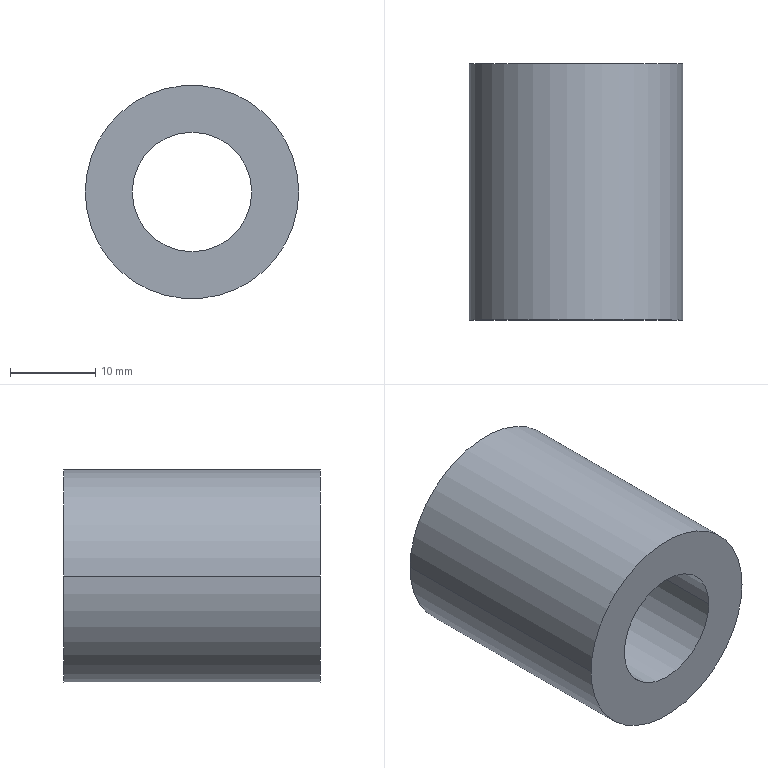Component | SolidWorks | UpperBushing-1 | 1 solid | 6 faces | box 25 x 30 x 25 mm | volume 10108 mm3 | cylinder 4 | plane 2 | commonest cylinder face diameters 14 x2 25 x2
build123d program:
from build123d import *

# Parameters (mm, degrees)
SKETCH1_R           = 12.5
SKETCH1_R_2         = 7
BOSS_EXTRUDE1_DEPTH = 30


with BuildPart() as part:
    # Sketch1 → Boss-Extrude1 (new body)
    with BuildSketch(Plane.XY):
        with Locations((-75, 62.5)):
            Circle(SKETCH1_R)
        with Locations((-75, 62.5)):
            Circle(SKETCH1_R_2, mode=Mode.SUBTRACT)
    extrude(amount=-BOSS_EXTRUDE1_DEPTH)


solid = part.part

# Placed as in the assembly
solid = solid.moved(Location((0, 170.565, -125), (90, 0, 0)))
STEP:
#1=CARTESIAN_POINT('',(-3.228,6.715,-2.461));
#2=VERTEX_POINT('',#1);
#3=CARTESIAN_POINT('',(-2.677,6.715,-2.461));
#4=VERTEX_POINT('',#3);
#5=CARTESIAN_POINT('',(-2.953,6.715,-2.461));
#6=DIRECTION('',(0.,1.,0.));
#7=DIRECTION('',(1.,0.,0.));
#8=AXIS2_PLACEMENT_3D('',#5,#6,#7);
#9=CIRCLE('',#8,0.2756);
#10=EDGE_CURVE('',#2,#4,#9,.T.);
#11=ORIENTED_EDGE('',*,*,#10,.F.);
#12=CARTESIAN_POINT('',(-3.228,7.896,-2.461));
#13=VERTEX_POINT('',#12);
#14=CARTESIAN_POINT('',(-3.228,6.715,-2.461));
#15=DIRECTION('',(0.,1.,0.));
#16=VECTOR('',#15,39.37);
#17=LINE('',#14,#16);
#18=EDGE_CURVE('',#2,#13,#17,.T.);
#19=ORIENTED_EDGE('',*,*,#18,.T.);
#20=CARTESIAN_POINT('',(-2.677,7.896,-2.461));
#21=VERTEX_POINT('',#20);
#22=CARTESIAN_POINT('',(-2.953,7.896,-2.461));
#23=DIRECTION('',(0.,1.,0.));
#24=DIRECTION('',(1.,0.,0.));
#25=AXIS2_PLACEMENT_3D('',#22,#23,#24);
#26=CIRCLE('',#25,0.2756);
#27=EDGE_CURVE('',#13,#21,#26,.T.);
#28=ORIENTED_EDGE('',*,*,#27,.T.);
#29=CARTESIAN_POINT('',(-2.677,6.715,-2.461));
#30=DIRECTION('',(0.,1.,0.));
#31=VECTOR('',#30,39.37);
#32=LINE('',#29,#31);
#33=EDGE_CURVE('',#4,#21,#32,.T.);
#34=ORIENTED_EDGE('',*,*,#33,.F.);
#35=EDGE_LOOP('',(#11,#19,#28,#34));
#36=FACE_OUTER_BOUND('',#35,.T.);
#37=CARTESIAN_POINT('',(-2.953,6.715,-2.461));
#38=DIRECTION('',(0.,1.,0.));
#39=DIRECTION('',(1.,0.,0.));
#40=AXIS2_PLACEMENT_3D('',#37,#38,#39);
#41=CYLINDRICAL_SURFACE('',#40,0.2756);
#42=ADVANCED_FACE('',(#36),#41,.F.);
#43=CARTESIAN_POINT('',(-2.461,6.715,-2.461));
#44=VERTEX_POINT('',#43);
#45=CARTESIAN_POINT('',(-3.445,6.715,-2.461));
#46=VERTEX_POINT('',#45);
#47=CARTESIAN_POINT('',(-2.953,6.715,-2.461));
#48=DIRECTION('',(0.,1.,0.));
#49=DIRECTION('',(1.,0.,0.));
#50=AXIS2_PLACEMENT_3D('',#47,#48,#49);
#51=CIRCLE('',#50,0.4921);
#52=EDGE_CURVE('',#44,#46,#51,.T.);
#53=ORIENTED_EDGE('',*,*,#52,.T.);
#54=CARTESIAN_POINT('',(-3.445,7.896,-2.461));
#55=VERTEX_POINT('',#54);
#56=CARTESIAN_POINT('',(-3.445,6.715,-2.461));
#57=DIRECTION('',(0.,1.,0.));
#58=VECTOR('',#57,39.37);
#59=LINE('',#56,#58);
#60=EDGE_CURVE('',#46,#55,#59,.T.);
#61=ORIENTED_EDGE('',*,*,#60,.T.);
#62=CARTESIAN_POINT('',(-2.461,7.896,-2.461));
#63=VERTEX_POINT('',#62);
#64=CARTESIAN_POINT('',(-2.953,7.896,-2.461));
#65=DIRECTION('',(0.,1.,0.));
#66=DIRECTION('',(1.,0.,0.));
#67=AXIS2_PLACEMENT_3D('',#64,#65,#66);
#68=CIRCLE('',#67,0.4921);
#69=EDGE_CURVE('',#63,#55,#68,.T.);
#70=ORIENTED_EDGE('',*,*,#69,.F.);
#71=CARTESIAN_POINT('',(-2.461,6.715,-2.461));
#72=DIRECTION('',(0.,1.,0.));
#73=VECTOR('',#72,39.37);
#74=LINE('',#71,#73);
#75=EDGE_CURVE('',#44,#63,#74,.T.);
#76=ORIENTED_EDGE('',*,*,#75,.F.);
#77=EDGE_LOOP('',(#53,#61,#70,#76));
#78=FACE_OUTER_BOUND('',#77,.T.);
#79=CARTESIAN_POINT('',(-2.953,6.715,-2.461));
#80=DIRECTION('',(0.,1.,0.));
#81=DIRECTION('',(1.,0.,0.));
#82=AXIS2_PLACEMENT_3D('',#79,#80,#81);
#83=CYLINDRICAL_SURFACE('',#82,0.4921);
#84=ADVANCED_FACE('',(#78),#83,.T.);
#85=ORIENTED_EDGE('',*,*,#60,.F.);
#86=CARTESIAN_POINT('',(-2.953,6.715,-2.461));
#87=DIRECTION('',(0.,1.,0.));
#88=DIRECTION('',(1.,0.,0.));
#89=AXIS2_PLACEMENT_3D('',#86,#87,#88);
#90=CIRCLE('',#89,0.4921);
#91=EDGE_CURVE('',#46,#44,#90,.T.);
#92=ORIENTED_EDGE('',*,*,#91,.T.);
#93=ORIENTED_EDGE('',*,*,#75,.T.);
#94=CARTESIAN_POINT('',(-2.953,7.896,-2.461));
#95=DIRECTION('',(0.,1.,0.));
#96=DIRECTION('',(1.,0.,0.));
#97=AXIS2_PLACEMENT_3D('',#94,#95,#96);
#98=CIRCLE('',#97,0.4921);
#99=EDGE_CURVE('',#55,#63,#98,.T.);
#100=ORIENTED_EDGE('',*,*,#99,.F.);
#101=EDGE_LOOP('',(#85,#92,#93,#100));
#102=FACE_OUTER_BOUND('',#101,.T.);
#103=CARTESIAN_POINT('',(-2.953,6.715,-2.461));
#104=DIRECTION('',(0.,1.,0.));
#105=DIRECTION('',(1.,0.,0.));
#106=AXIS2_PLACEMENT_3D('',#103,#104,#105);
#107=CYLINDRICAL_SURFACE('',#106,0.4921);
#108=ADVANCED_FACE('',(#102),#107,.T.);
#109=CARTESIAN_POINT('',(-2.953,6.715,-2.461));
#110=DIRECTION('',(0.,1.,0.));
#111=DIRECTION('',(1.,0.,0.));
#112=AXIS2_PLACEMENT_3D('',#109,#110,#111);
#113=CIRCLE('',#112,0.2756);
#114=EDGE_CURVE('',#4,#2,#113,.T.);
#115=ORIENTED_EDGE('',*,*,#114,.T.);
#116=ORIENTED_EDGE('',*,*,#10,.T.);
#117=EDGE_LOOP('',(#115,#116));
#118=FACE_BOUND('',#117,.T.);
#119=ORIENTED_EDGE('',*,*,#52,.F.);
#120=ORIENTED_EDGE('',*,*,#91,.F.);
#121=EDGE_LOOP('',(#119,#120));
#122=FACE_OUTER_BOUND('',#121,.T.);
#123=CARTESIAN_POINT('',(-2.953,6.715,-2.461));
#124=DIRECTION('',(0.,1.,0.));
#125=DIRECTION('',(1.,0.,0.));
#126=AXIS2_PLACEMENT_3D('',#123,#124,#125);
#127=PLANE('',#126);
#128=ADVANCED_FACE('',(#118,#122),#127,.F.);
#129=CARTESIAN_POINT('',(-2.953,7.896,-2.461));
#130=DIRECTION('',(0.,1.,0.));
#131=DIRECTION('',(1.,0.,0.));
#132=AXIS2_PLACEMENT_3D('',#129,#130,#131);
#133=CIRCLE('',#132,0.2756);
#134=EDGE_CURVE('',#21,#13,#133,.T.);
#135=ORIENTED_EDGE('',*,*,#134,.F.);
#136=ORIENTED_EDGE('',*,*,#27,.F.);
#137=EDGE_LOOP('',(#135,#136));
#138=FACE_BOUND('',#137,.T.);
#139=ORIENTED_EDGE('',*,*,#69,.T.);
#140=ORIENTED_EDGE('',*,*,#99,.T.);
#141=EDGE_LOOP('',(#139,#140));
#142=FACE_OUTER_BOUND('',#141,.T.);
#143=CARTESIAN_POINT('',(-2.953,7.896,-2.461));
#144=DIRECTION('',(0.,1.,0.));
#145=DIRECTION('',(1.,0.,0.));
#146=AXIS2_PLACEMENT_3D('',#143,#144,#145);
#147=PLANE('',#146);
#148=ADVANCED_FACE('',(#138,#142),#147,.T.);
#149=ORIENTED_EDGE('',*,*,#18,.F.);
#150=ORIENTED_EDGE('',*,*,#114,.F.);
#151=ORIENTED_EDGE('',*,*,#33,.T.);
#152=ORIENTED_EDGE('',*,*,#134,.T.);
#153=EDGE_LOOP('',(#149,#150,#151,#152));
#154=FACE_OUTER_BOUND('',#153,.T.);
#155=CARTESIAN_POINT('',(-2.953,6.715,-2.461));
#156=DIRECTION('',(0.,1.,0.));
#157=DIRECTION('',(1.,0.,0.));
#158=AXIS2_PLACEMENT_3D('',#155,#156,#157);
#159=CYLINDRICAL_SURFACE('',#158,0.2756);
#160=ADVANCED_FACE('',(#154),#159,.F.);
#161=CLOSED_SHELL('',(#42,#84,#108,#128,#148,#160));
#162=MANIFOLD_SOLID_BREP('',#161);
#163=CARTESIAN_POINT('',(0.,0.,0.));
#164=DIRECTION('',(0.,0.,1.));
#165=DIRECTION('',(1.,0.,0.));
#166=AXIS2_PLACEMENT_3D('',#163,#164,#165);
#167=(LENGTH_UNIT()NAMED_UNIT(*)SI_UNIT($,.METRE.));
#168=LENGTH_MEASURE_WITH_UNIT(LENGTH_MEASURE(0.0254),#167);
#169=DIMENSIONAL_EXPONENTS(1.,0.,0.,0.,0.,0.,0.);
#170=(CONVERSION_BASED_UNIT('',#168)LENGTH_UNIT()NAMED_UNIT(#169));
#171=UNCERTAINTY_MEASURE_WITH_UNIT(LENGTH_MEASURE(0.00001),#170,'','');
#172=(NAMED_UNIT(*)PLANE_ANGLE_UNIT()SI_UNIT($,.RADIAN.));
#173=(NAMED_UNIT(*)SI_UNIT($,.STERADIAN.)SOLID_ANGLE_UNIT());
#174=(GEOMETRIC_REPRESENTATION_CONTEXT(3)GLOBAL_UNCERTAINTY_ASSIGNED_CONTEXT((#171))GLOBAL_UNIT_ASSIGNED_CONTEXT((#170,#172,#173))REPRESENTATION_CONTEXT('',''));
#175=ADVANCED_BREP_SHAPE_REPRESENTATION('',(#162,#166),#174);
#176=COLOUR_RGB('',0.7922,0.8196,0.9333);
#177=FILL_AREA_STYLE_COLOUR('',#176);
#178=FILL_AREA_STYLE('',(#177));
#179=SURFACE_STYLE_FILL_AREA(#178);
#180=SURFACE_SIDE_STYLE('',(#179));
#181=SURFACE_STYLE_USAGE(.BOTH.,#180);
#182=PRESENTATION_STYLE_ASSIGNMENT((#181));
#183=STYLED_ITEM('',(#182),#162);
#184=(LENGTH_UNIT()NAMED_UNIT(*)SI_UNIT($,.METRE.));
#185=LENGTH_MEASURE_WITH_UNIT(LENGTH_MEASURE(0.0254),#184);
#186=DIMENSIONAL_EXPONENTS(1.,0.,0.,0.,0.,0.,0.);
#187=(CONVERSION_BASED_UNIT('',#185)LENGTH_UNIT()NAMED_UNIT(#186));
#188=UNCERTAINTY_MEASURE_WITH_UNIT(LENGTH_MEASURE(0.00001),#187,'','');
#189=(NAMED_UNIT(*)PLANE_ANGLE_UNIT()SI_UNIT($,.RADIAN.));
#190=(NAMED_UNIT(*)SI_UNIT($,.STERADIAN.)SOLID_ANGLE_UNIT());
#191=(GEOMETRIC_REPRESENTATION_CONTEXT(3)GLOBAL_UNCERTAINTY_ASSIGNED_CONTEXT((#188))GLOBAL_UNIT_ASSIGNED_CONTEXT((#187,#189,#190))REPRESENTATION_CONTEXT('',''));
#192=MECHANICAL_DESIGN_GEOMETRIC_PRESENTATION_REPRESENTATION('',(#183),#191);
#193=PRESENTATION_LAYER_ASSIGNMENT('','',(#183));